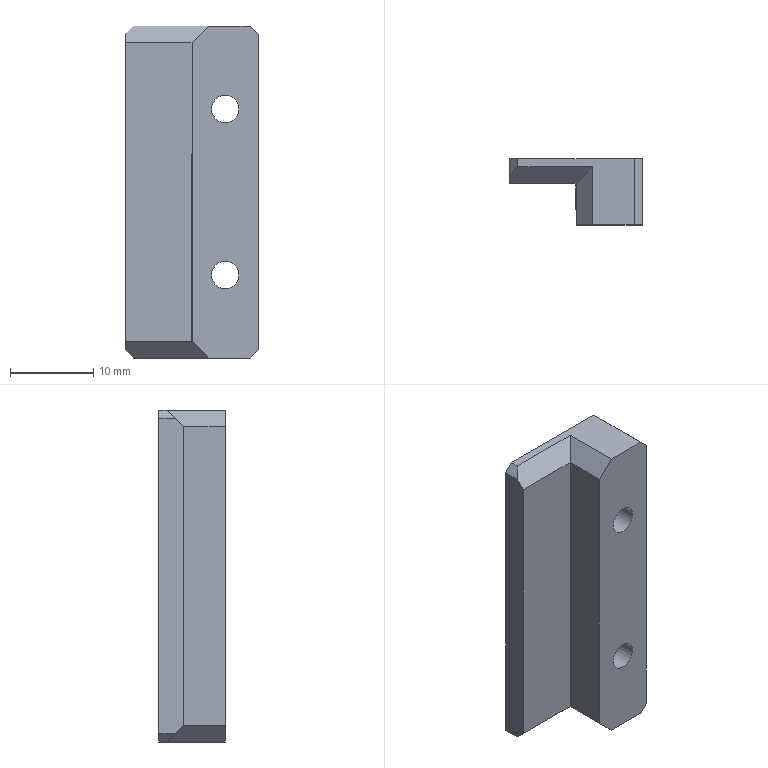Component | SolidWorks | J-TRD899MINI-2213-07DesiccantSlot-1 | 1 solid | 20 faces | box 16 x 8 x 40 mm | volume 3316 mm3 | plane 16 | cylinder 4 | commonest cylinder face diameters 3.3 x4 | material 6061
build123d program:
from build123d import *

# Parameters (mm, degrees)
BOSS_EXTRUDE1_DEPTH = 40
M4_TAPPED_HOLE1_D   = 3.3
CHAMFER1_SIZE       = 2
CHAMFER2_SIZE       = 1


with BuildPart() as part:
    # Sketch1 → Boss-Extrude1 (new body)
    with BuildSketch(Plane(origin=(0, 0, 0), x_dir=(0, 0, -1), z_dir=(1, 0, 0))):
        Polygon((0, 0), (8, 0), (8, 5), (16, 5), (16, 8), (0, 8), align=None)
    extrude(amount=BOSS_EXTRUDE1_DEPTH)

    # M4 Tapped Hole1 (through all)
    with Locations(Plane(origin=(0, 8, 0), x_dir=(1, 0, 0), z_dir=(0, 1, 0))):
        with Locations((10, 4), (30, 4)):
            Hole(M4_TAPPED_HOLE1_D / 2)

    # Chamfer1
    chamfer1_edges = [part.edges().sort_by_distance(p)[0] for p in [
        (40, 2.5, -8),
        (40, 5, -12),
        (0, 5, -12),
        (0, 2.5, -8),
    ]]
    chamfer(chamfer1_edges, length=CHAMFER1_SIZE)

    # Chamfer2
    chamfer2_edges = [part.edges().sort_by_distance(p)[0] for p in [
        (0, 7.5, -16),
        (40, 7.5, -16),
        (40, 4, 0),
        (0, 4, 0),
    ]]
    chamfer(chamfer2_edges, length=CHAMFER2_SIZE)


solid = part.part

# Placed as in the assembly
solid = solid.moved(Location((-45.663, -9.004, 169), (0, 90, 0)))
STEP:
#1=CARTESIAN_POINT('',(-2.02,-0.3545,6.26));
#2=VERTEX_POINT('',#1);
#3=CARTESIAN_POINT('',(-1.89,-0.3545,6.26));
#4=VERTEX_POINT('',#3);
#5=CARTESIAN_POINT('',(-1.955,-0.3545,6.26));
#6=DIRECTION('',(-0.,1.,0.));
#7=DIRECTION('',(1.,0.,0.));
#8=AXIS2_PLACEMENT_3D('',#5,#6,#7);
#9=CIRCLE('',#8,0.06496);
#10=EDGE_CURVE('',#2,#4,#9,.T.);
#11=ORIENTED_EDGE('',*,*,#10,.F.);
#12=CARTESIAN_POINT('',(-2.02,-0.03953,6.26));
#13=VERTEX_POINT('',#12);
#14=CARTESIAN_POINT('',(-2.02,-0.03953,6.26));
#15=DIRECTION('',(-0.,1.,0.));
#16=VECTOR('',#15,39.37);
#17=LINE('',#14,#16);
#18=EDGE_CURVE('',#2,#13,#17,.T.);
#19=ORIENTED_EDGE('',*,*,#18,.T.);
#20=CARTESIAN_POINT('',(-1.89,-0.03953,6.26));
#21=VERTEX_POINT('',#20);
#22=CARTESIAN_POINT('',(-1.955,-0.03953,6.26));
#23=DIRECTION('',(-0.,1.,0.));
#24=DIRECTION('',(1.,0.,0.));
#25=AXIS2_PLACEMENT_3D('',#22,#23,#24);
#26=CIRCLE('',#25,0.06496);
#27=EDGE_CURVE('',#13,#21,#26,.T.);
#28=ORIENTED_EDGE('',*,*,#27,.T.);
#29=CARTESIAN_POINT('',(-1.89,-0.03953,6.26));
#30=DIRECTION('',(-0.,1.,0.));
#31=VECTOR('',#30,39.37);
#32=LINE('',#29,#31);
#33=EDGE_CURVE('',#4,#21,#32,.T.);
#34=ORIENTED_EDGE('',*,*,#33,.F.);
#35=EDGE_LOOP('',(#11,#19,#28,#34));
#36=FACE_OUTER_BOUND('',#35,.T.);
#37=CARTESIAN_POINT('',(-1.955,-0.03953,6.26));
#38=DIRECTION('',(-0.,1.,0.));
#39=DIRECTION('',(1.,0.,0.));
#40=AXIS2_PLACEMENT_3D('',#37,#38,#39);
#41=CYLINDRICAL_SURFACE('',#40,0.06496);
#42=ADVANCED_FACE('',(#36),#41,.F.);
#43=CARTESIAN_POINT('',(-2.02,-0.3545,5.472));
#44=VERTEX_POINT('',#43);
#45=CARTESIAN_POINT('',(-1.89,-0.3545,5.472));
#46=VERTEX_POINT('',#45);
#47=CARTESIAN_POINT('',(-1.955,-0.3545,5.472));
#48=DIRECTION('',(-0.,1.,0.));
#49=DIRECTION('',(1.,0.,0.));
#50=AXIS2_PLACEMENT_3D('',#47,#48,#49);
#51=CIRCLE('',#50,0.06496);
#52=EDGE_CURVE('',#44,#46,#51,.T.);
#53=ORIENTED_EDGE('',*,*,#52,.F.);
#54=CARTESIAN_POINT('',(-2.02,-0.03953,5.472));
#55=VERTEX_POINT('',#54);
#56=CARTESIAN_POINT('',(-2.02,-0.03953,5.472));
#57=DIRECTION('',(-0.,1.,0.));
#58=VECTOR('',#57,39.37);
#59=LINE('',#56,#58);
#60=EDGE_CURVE('',#44,#55,#59,.T.);
#61=ORIENTED_EDGE('',*,*,#60,.T.);
#62=CARTESIAN_POINT('',(-1.89,-0.03953,5.472));
#63=VERTEX_POINT('',#62);
#64=CARTESIAN_POINT('',(-1.955,-0.03953,5.472));
#65=DIRECTION('',(-0.,1.,0.));
#66=DIRECTION('',(1.,0.,0.));
#67=AXIS2_PLACEMENT_3D('',#64,#65,#66);
#68=CIRCLE('',#67,0.06496);
#69=EDGE_CURVE('',#55,#63,#68,.T.);
#70=ORIENTED_EDGE('',*,*,#69,.T.);
#71=CARTESIAN_POINT('',(-1.89,-0.03953,5.472));
#72=DIRECTION('',(-0.,1.,0.));
#73=VECTOR('',#72,39.37);
#74=LINE('',#71,#73);
#75=EDGE_CURVE('',#46,#63,#74,.T.);
#76=ORIENTED_EDGE('',*,*,#75,.F.);
#77=EDGE_LOOP('',(#53,#61,#70,#76));
#78=FACE_OUTER_BOUND('',#77,.T.);
#79=CARTESIAN_POINT('',(-1.955,-0.03953,5.472));
#80=DIRECTION('',(-0.,1.,0.));
#81=DIRECTION('',(1.,0.,0.));
#82=AXIS2_PLACEMENT_3D('',#79,#80,#81);
#83=CYLINDRICAL_SURFACE('',#82,0.06496);
#84=ADVANCED_FACE('',(#78),#83,.F.);
#85=CARTESIAN_POINT('',(-1.798,-0.03953,5.118));
#86=VERTEX_POINT('',#85);
#87=CARTESIAN_POINT('',(-1.798,-0.03953,6.614));
#88=VERTEX_POINT('',#87);
#89=CARTESIAN_POINT('',(-1.798,-0.03953,5.079));
#90=DIRECTION('',(0.,-0.,1.));
#91=VECTOR('',#90,39.37);
#92=LINE('',#89,#91);
#93=EDGE_CURVE('',#86,#88,#92,.T.);
#94=ORIENTED_EDGE('',*,*,#93,.T.);
#95=CARTESIAN_POINT('',(-1.798,-0.3545,6.614));
#96=VERTEX_POINT('',#95);
#97=CARTESIAN_POINT('',(-1.798,-0.03953,6.614));
#98=DIRECTION('',(0.,-1.,-0.));
#99=VECTOR('',#98,39.37);
#100=LINE('',#97,#99);
#101=EDGE_CURVE('',#88,#96,#100,.T.);
#102=ORIENTED_EDGE('',*,*,#101,.T.);
#103=CARTESIAN_POINT('',(-1.798,-0.3545,5.118));
#104=VERTEX_POINT('',#103);
#105=CARTESIAN_POINT('',(-1.798,-0.3545,5.079));
#106=DIRECTION('',(0.,-0.,1.));
#107=VECTOR('',#106,39.37);
#108=LINE('',#105,#107);
#109=EDGE_CURVE('',#104,#96,#108,.T.);
#110=ORIENTED_EDGE('',*,*,#109,.F.);
#111=CARTESIAN_POINT('',(-1.798,-0.03953,5.118));
#112=DIRECTION('',(-0.,1.,0.));
#113=VECTOR('',#112,39.37);
#114=LINE('',#111,#113);
#115=EDGE_CURVE('',#104,#86,#114,.T.);
#116=ORIENTED_EDGE('',*,*,#115,.T.);
#117=EDGE_LOOP('',(#94,#102,#110,#116));
#118=FACE_OUTER_BOUND('',#117,.T.);
#119=CARTESIAN_POINT('',(-1.798,-0.03953,5.079));
#120=DIRECTION('',(-1.,-0.,0.));
#121=DIRECTION('',(-0.,1.,0.));
#122=AXIS2_PLACEMENT_3D('',#119,#120,#121);
#123=PLANE('',#122);
#124=ADVANCED_FACE('',(#118),#123,.F.);
#125=CARTESIAN_POINT('',(-1.955,-0.3545,6.26));
#126=DIRECTION('',(-0.,1.,0.));
#127=DIRECTION('',(1.,0.,0.));
#128=AXIS2_PLACEMENT_3D('',#125,#126,#127);
#129=CIRCLE('',#128,0.06496);
#130=EDGE_CURVE('',#4,#2,#129,.T.);
#131=ORIENTED_EDGE('',*,*,#130,.T.);
#132=ORIENTED_EDGE('',*,*,#10,.T.);
#133=EDGE_LOOP('',(#131,#132));
#134=FACE_BOUND('',#133,.T.);
#135=CARTESIAN_POINT('',(-1.955,-0.3545,5.472));
#136=DIRECTION('',(-0.,1.,0.));
#137=DIRECTION('',(1.,0.,0.));
#138=AXIS2_PLACEMENT_3D('',#135,#136,#137);
#139=CIRCLE('',#138,0.06496);
#140=EDGE_CURVE('',#46,#44,#139,.T.);
#141=ORIENTED_EDGE('',*,*,#140,.T.);
#142=ORIENTED_EDGE('',*,*,#52,.T.);
#143=EDGE_LOOP('',(#141,#142));
#144=FACE_BOUND('',#143,.T.);
#145=ORIENTED_EDGE('',*,*,#109,.T.);
#146=CARTESIAN_POINT('',(-1.837,-0.3545,6.654));
#147=VERTEX_POINT('',#146);
#148=CARTESIAN_POINT('',(-1.798,-0.3545,6.614));
#149=DIRECTION('',(-0.7071,-0.,0.7071));
#150=VECTOR('',#149,39.37);
#151=LINE('',#148,#150);
#152=EDGE_CURVE('',#96,#147,#151,.T.);
#153=ORIENTED_EDGE('',*,*,#152,.T.);
#154=CARTESIAN_POINT('',(-2.034,-0.3545,6.654));
#155=VERTEX_POINT('',#154);
#156=CARTESIAN_POINT('',(-1.798,-0.3545,6.654));
#157=DIRECTION('',(-1.,-0.,0.));
#158=VECTOR('',#157,39.37);
#159=LINE('',#156,#158);
#160=EDGE_CURVE('',#147,#155,#159,.T.);
#161=ORIENTED_EDGE('',*,*,#160,.T.);
#162=CARTESIAN_POINT('',(-2.113,-0.3545,6.575));
#163=VERTEX_POINT('',#162);
#164=CARTESIAN_POINT('',(-2.113,-0.3545,6.575));
#165=DIRECTION('',(-0.7071,-0.,-0.7071));
#166=VECTOR('',#165,39.37);
#167=LINE('',#164,#166);
#168=EDGE_CURVE('',#155,#163,#167,.T.);
#169=ORIENTED_EDGE('',*,*,#168,.T.);
#170=CARTESIAN_POINT('',(-2.113,-0.3545,5.157));
#171=VERTEX_POINT('',#170);
#172=CARTESIAN_POINT('',(-2.113,-0.3545,5.079));
#173=DIRECTION('',(0.,-0.,1.));
#174=VECTOR('',#173,39.37);
#175=LINE('',#172,#174);
#176=EDGE_CURVE('',#171,#163,#175,.T.);
#177=ORIENTED_EDGE('',*,*,#176,.F.);
#178=CARTESIAN_POINT('',(-2.034,-0.3545,5.079));
#179=VERTEX_POINT('',#178);
#180=CARTESIAN_POINT('',(-2.034,-0.3545,5.079));
#181=DIRECTION('',(0.7071,0.,-0.7071));
#182=VECTOR('',#181,39.37);
#183=LINE('',#180,#182);
#184=EDGE_CURVE('',#171,#179,#183,.T.);
#185=ORIENTED_EDGE('',*,*,#184,.T.);
#186=CARTESIAN_POINT('',(-1.837,-0.3545,5.079));
#187=VERTEX_POINT('',#186);
#188=CARTESIAN_POINT('',(-1.798,-0.3545,5.079));
#189=DIRECTION('',(-1.,-0.,0.));
#190=VECTOR('',#189,39.37);
#191=LINE('',#188,#190);
#192=EDGE_CURVE('',#187,#179,#191,.T.);
#193=ORIENTED_EDGE('',*,*,#192,.F.);
#194=CARTESIAN_POINT('',(-1.837,-0.3545,5.079));
#195=DIRECTION('',(0.7071,-0.,0.7071));
#196=VECTOR('',#195,39.37);
#197=LINE('',#194,#196);
#198=EDGE_CURVE('',#187,#104,#197,.T.);
#199=ORIENTED_EDGE('',*,*,#198,.T.);
#200=EDGE_LOOP('',(#145,#153,#161,#169,#177,#185,#193,#199));
#201=FACE_OUTER_BOUND('',#200,.T.);
#202=CARTESIAN_POINT('',(-1.798,-0.3545,5.079));
#203=DIRECTION('',(-0.,1.,0.));
#204=DIRECTION('',(1.,0.,-0.));
#205=AXIS2_PLACEMENT_3D('',#202,#203,#204);
#206=PLANE('',#205);
#207=ADVANCED_FACE('',(#134,#144,#201),#206,.F.);
#208=ORIENTED_EDGE('',*,*,#176,.T.);
#209=CARTESIAN_POINT('',(-2.113,-0.1576,6.575));
#210=VERTEX_POINT('',#209);
#211=CARTESIAN_POINT('',(-2.113,-0.3545,6.575));
#212=DIRECTION('',(-0.,1.,0.));
#213=VECTOR('',#212,39.37);
#214=LINE('',#211,#213);
#215=EDGE_CURVE('',#163,#210,#214,.T.);
#216=ORIENTED_EDGE('',*,*,#215,.T.);
#217=CARTESIAN_POINT('',(-2.113,-0.1576,5.157));
#218=VERTEX_POINT('',#217);
#219=CARTESIAN_POINT('',(-2.113,-0.1576,5.079));
#220=DIRECTION('',(0.,-0.,1.));
#221=VECTOR('',#220,39.37);
#222=LINE('',#219,#221);
#223=EDGE_CURVE('',#218,#210,#222,.T.);
#224=ORIENTED_EDGE('',*,*,#223,.F.);
#225=CARTESIAN_POINT('',(-2.113,-0.3545,5.157));
#226=DIRECTION('',(0.,-1.,-0.));
#227=VECTOR('',#226,39.37);
#228=LINE('',#225,#227);
#229=EDGE_CURVE('',#218,#171,#228,.T.);
#230=ORIENTED_EDGE('',*,*,#229,.T.);
#231=EDGE_LOOP('',(#208,#216,#224,#230));
#232=FACE_OUTER_BOUND('',#231,.T.);
#233=CARTESIAN_POINT('',(-2.113,-0.3545,5.079));
#234=DIRECTION('',(1.,0.,-0.));
#235=DIRECTION('',(-0.,0.,-1.));
#236=AXIS2_PLACEMENT_3D('',#233,#234,#235);
#237=PLANE('',#236);
#238=ADVANCED_FACE('',(#232),#237,.F.);
#239=ORIENTED_EDGE('',*,*,#223,.T.);
#240=CARTESIAN_POINT('',(-2.428,-0.1576,6.575));
#241=VERTEX_POINT('',#240);
#242=CARTESIAN_POINT('',(-2.113,-0.1576,6.575));
#243=DIRECTION('',(-1.,-0.,0.));
#244=VECTOR('',#243,39.37);
#245=LINE('',#242,#244);
#246=EDGE_CURVE('',#210,#241,#245,.T.);
#247=ORIENTED_EDGE('',*,*,#246,.T.);
#248=CARTESIAN_POINT('',(-2.428,-0.1576,5.157));
#249=VERTEX_POINT('',#248);
#250=CARTESIAN_POINT('',(-2.428,-0.1576,5.079));
#251=DIRECTION('',(0.,-0.,1.));
#252=VECTOR('',#251,39.37);
#253=LINE('',#250,#252);
#254=EDGE_CURVE('',#249,#241,#253,.T.);
#255=ORIENTED_EDGE('',*,*,#254,.F.);
#256=CARTESIAN_POINT('',(-2.113,-0.1576,5.157));
#257=DIRECTION('',(1.,0.,-0.));
#258=VECTOR('',#257,39.37);
#259=LINE('',#256,#258);
#260=EDGE_CURVE('',#249,#218,#259,.T.);
#261=ORIENTED_EDGE('',*,*,#260,.T.);
#262=EDGE_LOOP('',(#239,#247,#255,#261));
#263=FACE_OUTER_BOUND('',#262,.T.);
#264=CARTESIAN_POINT('',(-2.113,-0.1576,5.079));
#265=DIRECTION('',(-0.,1.,0.));
#266=DIRECTION('',(1.,0.,-0.));
#267=AXIS2_PLACEMENT_3D('',#264,#265,#266);
#268=PLANE('',#267);
#269=ADVANCED_FACE('',(#263),#268,.F.);
#270=CARTESIAN_POINT('',(-2.428,-0.1183,6.614));
#271=VERTEX_POINT('',#270);
#272=CARTESIAN_POINT('',(-2.428,-0.1576,6.575));
#273=DIRECTION('',(-0.,0.7071,0.7071));
#274=VECTOR('',#273,39.37);
#275=LINE('',#272,#274);
#276=EDGE_CURVE('',#241,#271,#275,.T.);
#277=ORIENTED_EDGE('',*,*,#276,.T.);
#278=CARTESIAN_POINT('',(-2.428,-0.03953,6.614));
#279=VERTEX_POINT('',#278);
#280=CARTESIAN_POINT('',(-2.428,-0.1576,6.614));
#281=DIRECTION('',(-0.,1.,0.));
#282=VECTOR('',#281,39.37);
#283=LINE('',#280,#282);
#284=EDGE_CURVE('',#271,#279,#283,.T.);
#285=ORIENTED_EDGE('',*,*,#284,.T.);
#286=CARTESIAN_POINT('',(-2.428,-0.03953,5.118));
#287=VERTEX_POINT('',#286);
#288=CARTESIAN_POINT('',(-2.428,-0.03953,5.079));
#289=DIRECTION('',(0.,-0.,1.));
#290=VECTOR('',#289,39.37);
#291=LINE('',#288,#290);
#292=EDGE_CURVE('',#287,#279,#291,.T.);
#293=ORIENTED_EDGE('',*,*,#292,.F.);
#294=CARTESIAN_POINT('',(-2.428,-0.1183,5.118));
#295=VERTEX_POINT('',#294);
#296=CARTESIAN_POINT('',(-2.428,-0.0789,5.118));
#297=DIRECTION('',(0.,-1.,-0.));
#298=VECTOR('',#297,39.37);
#299=LINE('',#296,#298);
#300=EDGE_CURVE('',#287,#295,#299,.T.);
#301=ORIENTED_EDGE('',*,*,#300,.T.);
#302=CARTESIAN_POINT('',(-2.428,-0.0789,5.079));
#303=DIRECTION('',(0.,-0.7071,0.7071));
#304=VECTOR('',#303,39.37);
#305=LINE('',#302,#304);
#306=EDGE_CURVE('',#295,#249,#305,.T.);
#307=ORIENTED_EDGE('',*,*,#306,.T.);
#308=ORIENTED_EDGE('',*,*,#254,.T.);
#309=EDGE_LOOP('',(#277,#285,#293,#301,#307,#308));
#310=FACE_OUTER_BOUND('',#309,.T.);
#311=CARTESIAN_POINT('',(-2.428,-0.1576,5.079));
#312=DIRECTION('',(1.,0.,-0.));
#313=DIRECTION('',(-0.,0.,-1.));
#314=AXIS2_PLACEMENT_3D('',#311,#312,#313);
#315=PLANE('',#314);
#316=ADVANCED_FACE('',(#310),#315,.F.);
#317=CARTESIAN_POINT('',(-1.955,-0.03953,6.26));
#318=DIRECTION('',(-0.,1.,0.));
#319=DIRECTION('',(1.,0.,0.));
#320=AXIS2_PLACEMENT_3D('',#317,#318,#319);
#321=CIRCLE('',#320,0.06496);
#322=EDGE_CURVE('',#21,#13,#321,.T.);
#323=ORIENTED_EDGE('',*,*,#322,.F.);
#324=ORIENTED_EDGE('',*,*,#27,.F.);
#325=EDGE_LOOP('',(#323,#324));
#326=FACE_BOUND('',#325,.T.);
#327=CARTESIAN_POINT('',(-1.955,-0.03953,5.472));
#328=DIRECTION('',(-0.,1.,0.));
#329=DIRECTION('',(1.,0.,0.));
#330=AXIS2_PLACEMENT_3D('',#327,#328,#329);
#331=CIRCLE('',#330,0.06496);
#332=EDGE_CURVE('',#63,#55,#331,.T.);
#333=ORIENTED_EDGE('',*,*,#332,.F.);
#334=ORIENTED_EDGE('',*,*,#69,.F.);
#335=EDGE_LOOP('',(#333,#334));
#336=FACE_BOUND('',#335,.T.);
#337=ORIENTED_EDGE('',*,*,#292,.T.);
#338=CARTESIAN_POINT('',(-2.388,-0.03953,6.654));
#339=VERTEX_POINT('',#338);
#340=CARTESIAN_POINT('',(-2.428,-0.03953,6.614));
#341=DIRECTION('',(0.7071,-0.,0.7071));
#342=VECTOR('',#341,39.37);
#343=LINE('',#340,#342);
#344=EDGE_CURVE('',#279,#339,#343,.T.);
#345=ORIENTED_EDGE('',*,*,#344,.T.);
#346=CARTESIAN_POINT('',(-1.837,-0.03953,6.654));
#347=VERTEX_POINT('',#346);
#348=CARTESIAN_POINT('',(-2.428,-0.03953,6.654));
#349=DIRECTION('',(1.,0.,-0.));
#350=VECTOR('',#349,39.37);
#351=LINE('',#348,#350);
#352=EDGE_CURVE('',#339,#347,#351,.T.);
#353=ORIENTED_EDGE('',*,*,#352,.T.);
#354=CARTESIAN_POINT('',(-1.798,-0.03953,6.614));
#355=DIRECTION('',(0.7071,0.,-0.7071));
#356=VECTOR('',#355,39.37);
#357=LINE('',#354,#356);
#358=EDGE_CURVE('',#347,#88,#357,.T.);
#359=ORIENTED_EDGE('',*,*,#358,.T.);
#360=ORIENTED_EDGE('',*,*,#93,.F.);
#361=CARTESIAN_POINT('',(-1.837,-0.03953,5.079));
#362=VERTEX_POINT('',#361);
#363=CARTESIAN_POINT('',(-1.837,-0.03953,5.079));
#364=DIRECTION('',(-0.7071,0.,-0.7071));
#365=VECTOR('',#364,39.37);
#366=LINE('',#363,#365);
#367=EDGE_CURVE('',#86,#362,#366,.T.);
#368=ORIENTED_EDGE('',*,*,#367,.T.);
#369=CARTESIAN_POINT('',(-2.388,-0.03953,5.079));
#370=VERTEX_POINT('',#369);
#371=CARTESIAN_POINT('',(-2.428,-0.03953,5.079));
#372=DIRECTION('',(1.,0.,-0.));
#373=VECTOR('',#372,39.37);
#374=LINE('',#371,#373);
#375=EDGE_CURVE('',#370,#362,#374,.T.);
#376=ORIENTED_EDGE('',*,*,#375,.F.);
#377=CARTESIAN_POINT('',(-2.388,-0.03953,5.079));
#378=DIRECTION('',(-0.7071,-0.,0.7071));
#379=VECTOR('',#378,39.37);
#380=LINE('',#377,#379);
#381=EDGE_CURVE('',#370,#287,#380,.T.);
#382=ORIENTED_EDGE('',*,*,#381,.T.);
#383=EDGE_LOOP('',(#337,#345,#353,#359,#360,#368,#376,#382));
#384=FACE_OUTER_BOUND('',#383,.T.);
#385=CARTESIAN_POINT('',(-2.428,-0.03953,5.079));
#386=DIRECTION('',(0.,-1.,-0.));
#387=DIRECTION('',(-1.,-0.,0.));
#388=AXIS2_PLACEMENT_3D('',#385,#386,#387);
#389=PLANE('',#388);
#390=ADVANCED_FACE('',(#326,#336,#384),#389,.F.);
#391=CARTESIAN_POINT('',(-2.034,-0.0789,5.079));
#392=VERTEX_POINT('',#391);
#393=CARTESIAN_POINT('',(-2.388,-0.0789,5.079));
#394=VERTEX_POINT('',#393);
#395=CARTESIAN_POINT('',(-2.428,-0.0789,5.079));
#396=DIRECTION('',(-1.,-0.,0.));
#397=VECTOR('',#396,39.37);
#398=LINE('',#395,#397);
#399=EDGE_CURVE('',#392,#394,#398,.T.);
#400=ORIENTED_EDGE('',*,*,#399,.T.);
#401=CARTESIAN_POINT('',(-2.388,-0.03953,5.079));
#402=DIRECTION('',(-0.,1.,0.));
#403=VECTOR('',#402,39.37);
#404=LINE('',#401,#403);
#405=EDGE_CURVE('',#394,#370,#404,.T.);
#406=ORIENTED_EDGE('',*,*,#405,.T.);
#407=ORIENTED_EDGE('',*,*,#375,.T.);
#408=CARTESIAN_POINT('',(-1.837,-0.3545,5.079));
#409=DIRECTION('',(0.,-1.,-0.));
#410=VECTOR('',#409,39.37);
#411=LINE('',#408,#410);
#412=EDGE_CURVE('',#362,#187,#411,.T.);
#413=ORIENTED_EDGE('',*,*,#412,.T.);
#414=ORIENTED_EDGE('',*,*,#192,.T.);
#415=CARTESIAN_POINT('',(-2.034,-0.1576,5.079));
#416=DIRECTION('',(-0.,1.,0.));
#417=VECTOR('',#416,39.37);
#418=LINE('',#415,#417);
#419=EDGE_CURVE('',#179,#392,#418,.T.);
#420=ORIENTED_EDGE('',*,*,#419,.T.);
#421=EDGE_LOOP('',(#400,#406,#407,#413,#414,#420));
#422=FACE_OUTER_BOUND('',#421,.T.);
#423=CARTESIAN_POINT('',(-1.798,-0.3545,5.079));
#424=DIRECTION('',(-0.,0.,-1.));
#425=DIRECTION('',(-1.,-0.,0.));
#426=AXIS2_PLACEMENT_3D('',#423,#424,#425);
#427=PLANE('',#426);
#428=ADVANCED_FACE('',(#422),#427,.T.);
#429=ORIENTED_EDGE('',*,*,#352,.F.);
#430=CARTESIAN_POINT('',(-2.388,-0.0789,6.654));
#431=VERTEX_POINT('',#430);
#432=CARTESIAN_POINT('',(-2.388,-0.3545,6.654));
#433=DIRECTION('',(0.,-1.,-0.));
#434=VECTOR('',#433,39.37);
#435=LINE('',#432,#434);
#436=EDGE_CURVE('',#339,#431,#435,.T.);
#437=ORIENTED_EDGE('',*,*,#436,.T.);
#438=CARTESIAN_POINT('',(-2.034,-0.0789,6.654));
#439=VERTEX_POINT('',#438);
#440=CARTESIAN_POINT('',(-1.798,-0.0789,6.654));
#441=DIRECTION('',(1.,0.,-0.));
#442=VECTOR('',#441,39.37);
#443=LINE('',#440,#442);
#444=EDGE_CURVE('',#431,#439,#443,.T.);
#445=ORIENTED_EDGE('',*,*,#444,.T.);
#446=CARTESIAN_POINT('',(-2.034,-0.3545,6.654));
#447=DIRECTION('',(0.,-1.,-0.));
#448=VECTOR('',#447,39.37);
#449=LINE('',#446,#448);
#450=EDGE_CURVE('',#439,#155,#449,.T.);
#451=ORIENTED_EDGE('',*,*,#450,.T.);
#452=ORIENTED_EDGE('',*,*,#160,.F.);
#453=CARTESIAN_POINT('',(-1.837,-0.3545,6.654));
#454=DIRECTION('',(-0.,1.,0.));
#455=VECTOR('',#454,39.37);
#456=LINE('',#453,#455);
#457=EDGE_CURVE('',#147,#347,#456,.T.);
#458=ORIENTED_EDGE('',*,*,#457,.T.);
#459=EDGE_LOOP('',(#429,#437,#445,#451,#452,#458));
#460=FACE_OUTER_BOUND('',#459,.T.);
#461=CARTESIAN_POINT('',(-1.798,-0.3545,6.654));
#462=DIRECTION('',(-0.,0.,-1.));
#463=DIRECTION('',(-1.,-0.,0.));
#464=AXIS2_PLACEMENT_3D('',#461,#462,#463);
#465=PLANE('',#464);
#466=ADVANCED_FACE('',(#460),#465,.F.);
#467=ORIENTED_EDGE('',*,*,#60,.F.);
#468=ORIENTED_EDGE('',*,*,#140,.F.);
#469=ORIENTED_EDGE('',*,*,#75,.T.);
#470=ORIENTED_EDGE('',*,*,#332,.T.);
#471=EDGE_LOOP('',(#467,#468,#469,#470));
#472=FACE_OUTER_BOUND('',#471,.T.);
#473=CARTESIAN_POINT('',(-1.955,-0.03953,5.472));
#474=DIRECTION('',(-0.,1.,0.));
#475=DIRECTION('',(1.,0.,0.));
#476=AXIS2_PLACEMENT_3D('',#473,#474,#475);
#477=CYLINDRICAL_SURFACE('',#476,0.06496);
#478=ADVANCED_FACE('',(#472),#477,.F.);
#479=ORIENTED_EDGE('',*,*,#18,.F.);
#480=ORIENTED_EDGE('',*,*,#130,.F.);
#481=ORIENTED_EDGE('',*,*,#33,.T.);
#482=ORIENTED_EDGE('',*,*,#322,.T.);
#483=EDGE_LOOP('',(#479,#480,#481,#482));
#484=FACE_OUTER_BOUND('',#483,.T.);
#485=CARTESIAN_POINT('',(-1.955,-0.03953,6.26));
#486=DIRECTION('',(-0.,1.,0.));
#487=DIRECTION('',(1.,0.,0.));
#488=AXIS2_PLACEMENT_3D('',#485,#486,#487);
#489=CYLINDRICAL_SURFACE('',#488,0.06496);
#490=ADVANCED_FACE('',(#484),#489,.F.);
#491=ORIENTED_EDGE('',*,*,#168,.F.);
#492=ORIENTED_EDGE('',*,*,#450,.F.);
#493=CARTESIAN_POINT('',(-2.113,-0.1576,6.575));
#494=DIRECTION('',(0.5774,0.5774,0.5774));
#495=VECTOR('',#494,39.37);
#496=LINE('',#493,#495);
#497=EDGE_CURVE('',#210,#439,#496,.T.);
#498=ORIENTED_EDGE('',*,*,#497,.F.);
#499=ORIENTED_EDGE('',*,*,#215,.F.);
#500=EDGE_LOOP('',(#491,#492,#498,#499));
#501=FACE_OUTER_BOUND('',#500,.T.);
#502=CARTESIAN_POINT('',(-2.113,-0.3545,6.575));
#503=DIRECTION('',(0.7071,0.,-0.7071));
#504=DIRECTION('',(-0.,1.,0.));
#505=AXIS2_PLACEMENT_3D('',#502,#503,#504);
#506=PLANE('',#505);
#507=ADVANCED_FACE('',(#501),#506,.F.);
#508=ORIENTED_EDGE('',*,*,#444,.F.);
#509=CARTESIAN_POINT('',(-2.349,-0.03953,6.693));
#510=DIRECTION('',(-0.5774,-0.5774,-0.5774));
#511=VECTOR('',#510,39.37);
#512=LINE('',#509,#511);
#513=EDGE_CURVE('',#431,#271,#512,.T.);
#514=ORIENTED_EDGE('',*,*,#513,.T.);
#515=ORIENTED_EDGE('',*,*,#276,.F.);
#516=ORIENTED_EDGE('',*,*,#246,.F.);
#517=ORIENTED_EDGE('',*,*,#497,.T.);
#518=EDGE_LOOP('',(#508,#514,#515,#516,#517));
#519=FACE_OUTER_BOUND('',#518,.T.);
#520=CARTESIAN_POINT('',(-2.113,-0.1576,6.575));
#521=DIRECTION('',(-0.,0.7071,-0.7071));
#522=DIRECTION('',(-1.,-0.,0.));
#523=AXIS2_PLACEMENT_3D('',#520,#521,#522);
#524=PLANE('',#523);
#525=ADVANCED_FACE('',(#519),#524,.F.);
#526=ORIENTED_EDGE('',*,*,#306,.F.);
#527=CARTESIAN_POINT('',(-2.191,0.118,4.882));
#528=DIRECTION('',(0.5774,0.5774,-0.5774));
#529=VECTOR('',#528,39.37);
#530=LINE('',#527,#529);
#531=EDGE_CURVE('',#295,#394,#530,.T.);
#532=ORIENTED_EDGE('',*,*,#531,.T.);
#533=ORIENTED_EDGE('',*,*,#399,.F.);
#534=CARTESIAN_POINT('',(-2.126,-0.1708,5.171));
#535=DIRECTION('',(0.5774,0.5774,-0.5774));
#536=VECTOR('',#535,39.37);
#537=LINE('',#534,#536);
#538=EDGE_CURVE('',#218,#392,#537,.T.);
#539=ORIENTED_EDGE('',*,*,#538,.F.);
#540=ORIENTED_EDGE('',*,*,#260,.F.);
#541=EDGE_LOOP('',(#526,#532,#533,#539,#540));
#542=FACE_OUTER_BOUND('',#541,.T.);
#543=CARTESIAN_POINT('',(-1.798,-0.0789,5.079));
#544=DIRECTION('',(0.,-0.7071,-0.7071));
#545=DIRECTION('',(1.,0.,-0.));
#546=AXIS2_PLACEMENT_3D('',#543,#544,#545);
#547=PLANE('',#546);
#548=ADVANCED_FACE('',(#542),#547,.T.);
#549=ORIENTED_EDGE('',*,*,#184,.F.);
#550=ORIENTED_EDGE('',*,*,#229,.F.);
#551=ORIENTED_EDGE('',*,*,#538,.T.);
#552=ORIENTED_EDGE('',*,*,#419,.F.);
#553=EDGE_LOOP('',(#549,#550,#551,#552));
#554=FACE_OUTER_BOUND('',#553,.T.);
#555=CARTESIAN_POINT('',(-2.034,-0.3545,5.079));
#556=DIRECTION('',(-0.7071,-0.,-0.7071));
#557=DIRECTION('',(0.,-1.,-0.));
#558=AXIS2_PLACEMENT_3D('',#555,#556,#557);
#559=PLANE('',#558);
#560=ADVANCED_FACE('',(#554),#559,.T.);
#561=ORIENTED_EDGE('',*,*,#513,.F.);
#562=ORIENTED_EDGE('',*,*,#436,.F.);
#563=ORIENTED_EDGE('',*,*,#344,.F.);
#564=ORIENTED_EDGE('',*,*,#284,.F.);
#565=EDGE_LOOP('',(#561,#562,#563,#564));
#566=FACE_OUTER_BOUND('',#565,.T.);
#567=CARTESIAN_POINT('',(-2.428,-0.1576,6.614));
#568=DIRECTION('',(0.7071,0.,-0.7071));
#569=DIRECTION('',(-0.,1.,0.));
#570=AXIS2_PLACEMENT_3D('',#567,#568,#569);
#571=PLANE('',#570);
#572=ADVANCED_FACE('',(#566),#571,.F.);
#573=ORIENTED_EDGE('',*,*,#531,.F.);
#574=ORIENTED_EDGE('',*,*,#300,.F.);
#575=ORIENTED_EDGE('',*,*,#381,.F.);
#576=ORIENTED_EDGE('',*,*,#405,.F.);
#577=EDGE_LOOP('',(#573,#574,#575,#576));
#578=FACE_OUTER_BOUND('',#577,.T.);
#579=CARTESIAN_POINT('',(-2.388,-0.3545,5.079));
#580=DIRECTION('',(-0.7071,-0.,-0.7071));
#581=DIRECTION('',(0.,-1.,-0.));
#582=AXIS2_PLACEMENT_3D('',#579,#580,#581);
#583=PLANE('',#582);
#584=ADVANCED_FACE('',(#578),#583,.T.);
#585=ORIENTED_EDGE('',*,*,#358,.F.);
#586=ORIENTED_EDGE('',*,*,#457,.F.);
#587=ORIENTED_EDGE('',*,*,#152,.F.);
#588=ORIENTED_EDGE('',*,*,#101,.F.);
#589=EDGE_LOOP('',(#585,#586,#587,#588));
#590=FACE_OUTER_BOUND('',#589,.T.);
#591=CARTESIAN_POINT('',(-1.798,-0.03953,6.614));
#592=DIRECTION('',(-0.7071,-0.,-0.7071));
#593=DIRECTION('',(0.,-1.,-0.));
#594=AXIS2_PLACEMENT_3D('',#591,#592,#593);
#595=PLANE('',#594);
#596=ADVANCED_FACE('',(#590),#595,.F.);
#597=ORIENTED_EDGE('',*,*,#367,.F.);
#598=ORIENTED_EDGE('',*,*,#115,.F.);
#599=ORIENTED_EDGE('',*,*,#198,.F.);
#600=ORIENTED_EDGE('',*,*,#412,.F.);
#601=EDGE_LOOP('',(#597,#598,#599,#600));
#602=FACE_OUTER_BOUND('',#601,.T.);
#603=CARTESIAN_POINT('',(-1.837,-0.3545,5.079));
#604=DIRECTION('',(0.7071,0.,-0.7071));
#605=DIRECTION('',(-0.,1.,0.));
#606=AXIS2_PLACEMENT_3D('',#603,#604,#605);
#607=PLANE('',#606);
#608=ADVANCED_FACE('',(#602),#607,.T.);
#609=CLOSED_SHELL('',(#42,#84,#124,#207,#238,#269,#316,#390,#428,#466,#478,#490,#507,#525,#548,#560,#572,#584,#596,#608));
#610=MANIFOLD_SOLID_BREP('',#609);
#611=CARTESIAN_POINT('',(0.,0.,0.));
#612=DIRECTION('',(0.,0.,1.));
#613=DIRECTION('',(1.,0.,0.));
#614=AXIS2_PLACEMENT_3D('',#611,#612,#613);
#615=(LENGTH_UNIT()NAMED_UNIT(*)SI_UNIT($,.METRE.));
#616=LENGTH_MEASURE_WITH_UNIT(LENGTH_MEASURE(0.0254),#615);
#617=DIMENSIONAL_EXPONENTS(1.,0.,0.,0.,0.,0.,0.);
#618=(CONVERSION_BASED_UNIT('',#616)LENGTH_UNIT()NAMED_UNIT(#617));
#619=UNCERTAINTY_MEASURE_WITH_UNIT(LENGTH_MEASURE(0.00001),#618,'','');
#620=(NAMED_UNIT(*)PLANE_ANGLE_UNIT()SI_UNIT($,.RADIAN.));
#621=(NAMED_UNIT(*)SI_UNIT($,.STERADIAN.)SOLID_ANGLE_UNIT());
#622=(GEOMETRIC_REPRESENTATION_CONTEXT(3)GLOBAL_UNCERTAINTY_ASSIGNED_CONTEXT((#619))GLOBAL_UNIT_ASSIGNED_CONTEXT((#618,#620,#621))REPRESENTATION_CONTEXT('',''));
#623=ADVANCED_BREP_SHAPE_REPRESENTATION('',(#610,#614),#622);
#624=COLOUR_RGB('',0.7922,0.8196,0.9333);
#625=FILL_AREA_STYLE_COLOUR('',#624);
#626=FILL_AREA_STYLE('',(#625));
#627=SURFACE_STYLE_FILL_AREA(#626);
#628=SURFACE_SIDE_STYLE('',(#627));
#629=SURFACE_STYLE_USAGE(.BOTH.,#628);
#630=PRESENTATION_STYLE_ASSIGNMENT((#629));
#631=STYLED_ITEM('',(#630),#610);
#632=(LENGTH_UNIT()NAMED_UNIT(*)SI_UNIT($,.METRE.));
#633=LENGTH_MEASURE_WITH_UNIT(LENGTH_MEASURE(0.0254),#632);
#634=DIMENSIONAL_EXPONENTS(1.,0.,0.,0.,0.,0.,0.);
#635=(CONVERSION_BASED_UNIT('',#633)LENGTH_UNIT()NAMED_UNIT(#634));
#636=UNCERTAINTY_MEASURE_WITH_UNIT(LENGTH_MEASURE(0.00001),#635,'','');
#637=(NAMED_UNIT(*)PLANE_ANGLE_UNIT()SI_UNIT($,.RADIAN.));
#638=(NAMED_UNIT(*)SI_UNIT($,.STERADIAN.)SOLID_ANGLE_UNIT());
#639=(GEOMETRIC_REPRESENTATION_CONTEXT(3)GLOBAL_UNCERTAINTY_ASSIGNED_CONTEXT((#636))GLOBAL_UNIT_ASSIGNED_CONTEXT((#635,#637,#638))REPRESENTATION_CONTEXT('',''));
#640=MECHANICAL_DESIGN_GEOMETRIC_PRESENTATION_REPRESENTATION('',(#631),#639);
#641=PRESENTATION_LAYER_ASSIGNMENT('','',(#631));